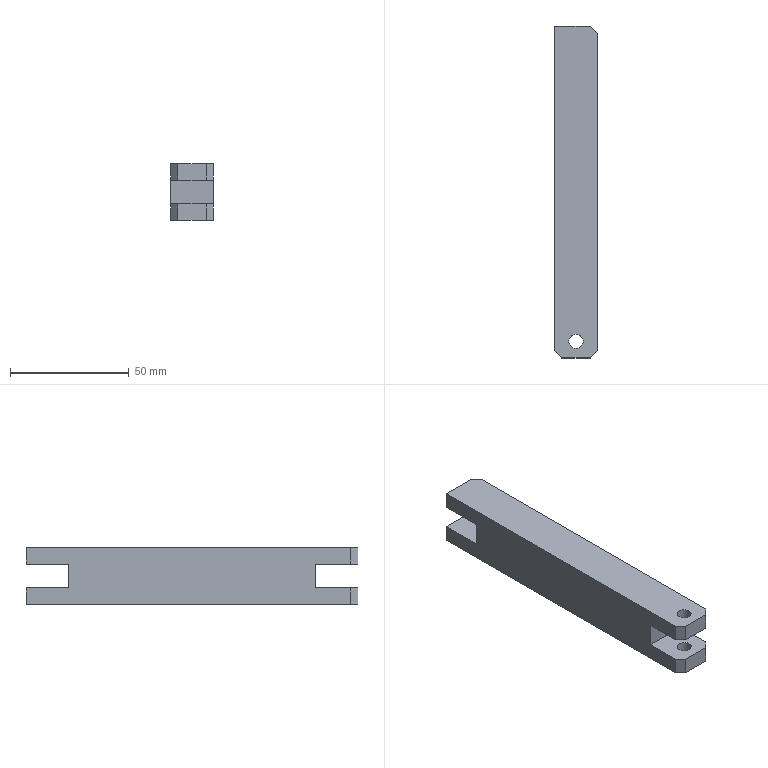Component | NX | CLAMP_PLATE | 1 solid | 22 faces | volume 53415 mm3 | plane 20 | cylinder 2 | commonest cylinder face diameters 6 x2